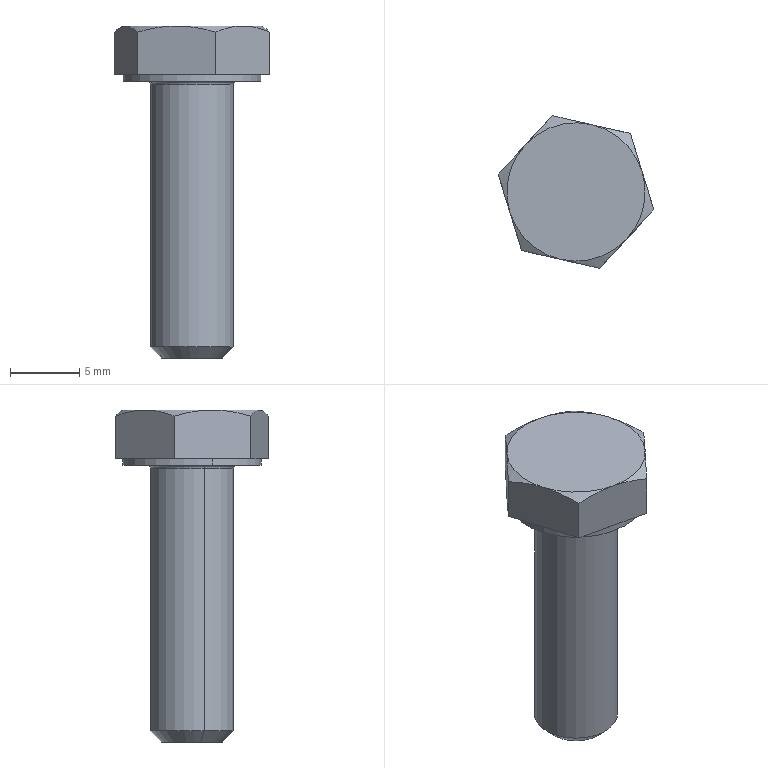Component | SolidWorks | GB_T5781-2000HexHeadBoltFullThreadCGradeM6_20-1 | 1 solid | 29 faces | box 11.25 x 11.04 x 24 mm | volume 902 mm3 | plane 15 | cone 8 | cylinder 4 | torus 2 | commonest cylinder face diameters 6 x2 10 x2 | material 8.8 Grade
STEP:
#1=COLOUR_RGB('',0.7922,0.8196,0.9333);
#2=FILL_AREA_STYLE_COLOUR('',#1);
#3=FILL_AREA_STYLE('',(#2));
#4=SURFACE_STYLE_FILL_AREA(#3);
#5=SURFACE_SIDE_STYLE('',(#4));
#6=SURFACE_STYLE_USAGE(.BOTH.,#5);
#7=PRESENTATION_STYLE_ASSIGNMENT((#6));
#8=CARTESIAN_POINT('',(4.631,0.8511,0.8248));
#9=VERTEX_POINT('',#8);
#10=CARTESIAN_POINT('',(4.857,0.9205,0.8248));
#11=VERTEX_POINT('',#10);
#12=CARTESIAN_POINT('',(4.744,0.8858,0.8248));
#13=DIRECTION('',(0.,0.,-1.));
#14=DIRECTION('',(0.9559,0.2937,0.));
#15=AXIS2_PLACEMENT_3D('',#12,#13,#14);
#16=CIRCLE('',#15,0.1181);
#17=EDGE_CURVE('',#9,#11,#16,.T.);
#18=ORIENTED_EDGE('',*,*,#17,.F.);
#19=CARTESIAN_POINT('',(4.622,0.8482,0.8346));
#20=VERTEX_POINT('',#19);
#21=CARTESIAN_POINT('',(4.622,0.8482,0.8248));
#22=DIRECTION('',(0.2937,-0.9559,0.));
#23=DIRECTION('',(0.9559,0.2937,0.));
#24=AXIS2_PLACEMENT_3D('',#21,#22,#23);
#25=CIRCLE('',#24,0.009843);
#26=EDGE_CURVE('',#9,#20,#25,.T.);
#27=ORIENTED_EDGE('',*,*,#26,.T.);
#28=CARTESIAN_POINT('',(4.866,0.9234,0.8346));
#29=VERTEX_POINT('',#28);
#30=CARTESIAN_POINT('',(4.744,0.8858,0.8346));
#31=DIRECTION('',(0.,0.,1.));
#32=DIRECTION('',(0.9559,0.2937,0.));
#33=AXIS2_PLACEMENT_3D('',#30,#31,#32);
#34=CIRCLE('',#33,0.128);
#35=EDGE_CURVE('',#29,#20,#34,.T.);
#36=ORIENTED_EDGE('',*,*,#35,.F.);
#37=CARTESIAN_POINT('',(4.866,0.9234,0.8248));
#38=DIRECTION('',(-0.2937,0.9559,0.));
#39=DIRECTION('',(-0.9559,-0.2937,0.));
#40=AXIS2_PLACEMENT_3D('',#37,#38,#39);
#41=CIRCLE('',#40,0.009843);
#42=EDGE_CURVE('',#11,#29,#41,.T.);
#43=ORIENTED_EDGE('',*,*,#42,.F.);
#44=EDGE_LOOP('',(#18,#27,#36,#43));
#45=FACE_OUTER_BOUND('',#44,.T.);
#46=CARTESIAN_POINT('',(4.744,0.8858,0.8248));
#47=DIRECTION('',(0.,0.,-1.));
#48=DIRECTION('',(0.9559,0.2937,0.));
#49=AXIS2_PLACEMENT_3D('',#46,#47,#48);
#50=TOROIDAL_SURFACE('',#49,0.128,0.009843);
#51=ADVANCED_FACE('',(#45),#50,.F.);
#52=CARTESIAN_POINT('',(4.827,0.9113,0.04724));
#53=VERTEX_POINT('',#52);
#54=CARTESIAN_POINT('',(4.661,0.8604,0.04724));
#55=VERTEX_POINT('',#54);
#56=CARTESIAN_POINT('',(4.744,0.8858,0.04724));
#57=DIRECTION('',(0.,0.,-1.));
#58=DIRECTION('',(-0.9559,-0.2937,0.));
#59=AXIS2_PLACEMENT_3D('',#56,#57,#58);
#60=CIRCLE('',#59,0.08661);
#61=EDGE_CURVE('',#53,#55,#60,.T.);
#62=ORIENTED_EDGE('',*,*,#61,.F.);
#63=CARTESIAN_POINT('',(4.857,0.9205,0.07874));
#64=VERTEX_POINT('',#63);
#65=CARTESIAN_POINT('',(4.857,0.9205,0.07874));
#66=DIRECTION('',(0.6759,0.2077,0.7071));
#67=VECTOR('',#66,39.37);
#68=LINE('',#65,#67);
#69=EDGE_CURVE('',#53,#64,#68,.T.);
#70=ORIENTED_EDGE('',*,*,#69,.T.);
#71=CARTESIAN_POINT('',(4.631,0.8511,0.07874));
#72=VERTEX_POINT('',#71);
#73=CARTESIAN_POINT('',(4.744,0.8858,0.07874));
#74=DIRECTION('',(0.,0.,1.));
#75=DIRECTION('',(-0.9559,-0.2937,0.));
#76=AXIS2_PLACEMENT_3D('',#73,#74,#75);
#77=CIRCLE('',#76,0.1181);
#78=EDGE_CURVE('',#72,#64,#77,.T.);
#79=ORIENTED_EDGE('',*,*,#78,.F.);
#80=CARTESIAN_POINT('',(4.631,0.8511,0.07874));
#81=DIRECTION('',(-0.6759,-0.2077,0.7071));
#82=VECTOR('',#81,39.37);
#83=LINE('',#80,#82);
#84=EDGE_CURVE('',#55,#72,#83,.T.);
#85=ORIENTED_EDGE('',*,*,#84,.F.);
#86=EDGE_LOOP('',(#62,#70,#79,#85));
#87=FACE_OUTER_BOUND('',#86,.T.);
#88=CARTESIAN_POINT('',(4.744,0.8858,0.07874));
#89=DIRECTION('',(0.,0.,1.));
#90=DIRECTION('',(-0.9559,-0.2937,0.));
#91=AXIS2_PLACEMENT_3D('',#88,#89,#90);
#92=CONICAL_SURFACE('',#91,0.1181,0.7854);
#93=ADVANCED_FACE('',(#87),#92,.T.);
#94=ORIENTED_EDGE('',*,*,#78,.T.);
#95=CARTESIAN_POINT('',(4.857,0.9205,0.9921));
#96=DIRECTION('',(0.,0.,1.));
#97=VECTOR('',#96,39.37);
#98=LINE('',#95,#97);
#99=EDGE_CURVE('',#64,#11,#98,.T.);
#100=ORIENTED_EDGE('',*,*,#99,.T.);
#101=CARTESIAN_POINT('',(4.744,0.8858,0.8248));
#102=DIRECTION('',(0.,0.,-1.));
#103=DIRECTION('',(0.9559,0.2937,0.));
#104=AXIS2_PLACEMENT_3D('',#101,#102,#103);
#105=CIRCLE('',#104,0.1181);
#106=EDGE_CURVE('',#11,#9,#105,.T.);
#107=ORIENTED_EDGE('',*,*,#106,.T.);
#108=CARTESIAN_POINT('',(4.631,0.8511,0.9921));
#109=DIRECTION('',(0.,0.,1.));
#110=VECTOR('',#109,39.37);
#111=LINE('',#108,#110);
#112=EDGE_CURVE('',#72,#9,#111,.T.);
#113=ORIENTED_EDGE('',*,*,#112,.F.);
#114=EDGE_LOOP('',(#94,#100,#107,#113));
#115=FACE_OUTER_BOUND('',#114,.T.);
#116=CARTESIAN_POINT('',(4.744,0.8858,0.9921));
#117=DIRECTION('',(0.,0.,1.));
#118=DIRECTION('',(-0.9559,-0.2937,0.));
#119=AXIS2_PLACEMENT_3D('',#116,#117,#118);
#120=CYLINDRICAL_SURFACE('',#119,0.1181);
#121=ADVANCED_FACE('',(#115),#120,.T.);
#122=CARTESIAN_POINT('',(4.932,0.9436,0.8346));
#123=VERTEX_POINT('',#122);
#124=CARTESIAN_POINT('',(4.556,0.828,0.8346));
#125=VERTEX_POINT('',#124);
#126=CARTESIAN_POINT('',(4.744,0.8858,0.8346));
#127=DIRECTION('',(0.,0.,-1.));
#128=DIRECTION('',(0.9559,0.2937,0.));
#129=AXIS2_PLACEMENT_3D('',#126,#127,#128);
#130=CIRCLE('',#129,0.1969);
#131=EDGE_CURVE('',#123,#125,#130,.T.);
#132=ORIENTED_EDGE('',*,*,#131,.F.);
#133=CARTESIAN_POINT('',(4.932,0.9436,0.8543));
#134=VERTEX_POINT('',#133);
#135=CARTESIAN_POINT('',(4.932,0.9436,0.9921));
#136=DIRECTION('',(0.,0.,1.));
#137=VECTOR('',#136,39.37);
#138=LINE('',#135,#137);
#139=EDGE_CURVE('',#123,#134,#138,.T.);
#140=ORIENTED_EDGE('',*,*,#139,.T.);
#141=CARTESIAN_POINT('',(4.888,0.7518,0.8543));
#142=VERTEX_POINT('',#141);
#143=CARTESIAN_POINT('',(4.744,0.8858,0.8543));
#144=DIRECTION('',(0.,0.,1.));
#145=DIRECTION('',(-0.9559,-0.2937,0.));
#146=AXIS2_PLACEMENT_3D('',#143,#144,#145);
#147=CIRCLE('',#146,0.1969);
#148=EDGE_CURVE('',#142,#134,#147,.T.);
#149=ORIENTED_EDGE('',*,*,#148,.F.);
#150=CARTESIAN_POINT('',(4.7,0.694,0.8543));
#151=VERTEX_POINT('',#150);
#152=CARTESIAN_POINT('',(4.744,0.8858,0.8543));
#153=DIRECTION('',(0.,0.,1.));
#154=DIRECTION('',(-0.9559,-0.2937,0.));
#155=AXIS2_PLACEMENT_3D('',#152,#153,#154);
#156=CIRCLE('',#155,0.1969);
#157=EDGE_CURVE('',#151,#142,#156,.T.);
#158=ORIENTED_EDGE('',*,*,#157,.F.);
#159=CARTESIAN_POINT('',(4.556,0.828,0.8543));
#160=VERTEX_POINT('',#159);
#161=CARTESIAN_POINT('',(4.744,0.8858,0.8543));
#162=DIRECTION('',(0.,0.,1.));
#163=DIRECTION('',(-0.9559,-0.2937,0.));
#164=AXIS2_PLACEMENT_3D('',#161,#162,#163);
#165=CIRCLE('',#164,0.1969);
#166=EDGE_CURVE('',#160,#151,#165,.T.);
#167=ORIENTED_EDGE('',*,*,#166,.F.);
#168=CARTESIAN_POINT('',(4.556,0.828,0.9921));
#169=DIRECTION('',(0.,0.,1.));
#170=VECTOR('',#169,39.37);
#171=LINE('',#168,#170);
#172=EDGE_CURVE('',#125,#160,#171,.T.);
#173=ORIENTED_EDGE('',*,*,#172,.F.);
#174=EDGE_LOOP('',(#132,#140,#149,#158,#167,#173));
#175=FACE_OUTER_BOUND('',#174,.T.);
#176=CARTESIAN_POINT('',(4.744,0.8858,0.9921));
#177=DIRECTION('',(0.,0.,1.));
#178=DIRECTION('',(-0.9559,-0.2937,0.));
#179=AXIS2_PLACEMENT_3D('',#176,#177,#178);
#180=CYLINDRICAL_SURFACE('',#179,0.1969);
#181=ADVANCED_FACE('',(#175),#180,.T.);
#182=CARTESIAN_POINT('',(4.965,0.835,0.8543));
#183=VERTEX_POINT('',#182);
#184=CARTESIAN_POINT('',(4.965,0.835,0.8543));
#185=DIRECTION('',(-0.681,-0.7323,0.));
#186=VECTOR('',#185,39.37);
#187=LINE('',#184,#186);
#188=EDGE_CURVE('',#183,#142,#187,.T.);
#189=ORIENTED_EDGE('',*,*,#188,.F.);
#190=CARTESIAN_POINT('',(4.965,0.835,0.9745));
#191=VERTEX_POINT('',#190);
#192=CARTESIAN_POINT('',(4.965,0.835,0.8346));
#193=DIRECTION('',(0.,0.,1.));
#194=VECTOR('',#193,39.37);
#195=LINE('',#192,#194);
#196=EDGE_CURVE('',#183,#191,#195,.T.);
#197=ORIENTED_EDGE('',*,*,#196,.T.);
#198=CARTESIAN_POINT('',(4.888,0.7518,0.9921));
#199=VERTEX_POINT('',#198);
#200=CARTESIAN_POINT('',(4.888,0.7518,0.9921));
#201=CARTESIAN_POINT('',(4.895,0.7588,0.9921));
#202=CARTESIAN_POINT('',(4.901,0.7659,0.9917));
#203=CARTESIAN_POINT('',(4.914,0.78,0.9901));
#204=CARTESIAN_POINT('',(4.921,0.7869,0.9889));
#205=CARTESIAN_POINT('',(4.94,0.8077,0.9843));
#206=CARTESIAN_POINT('',(4.953,0.8214,0.9799));
#207=CARTESIAN_POINT('',(4.965,0.835,0.9745));
#208=B_SPLINE_CURVE_WITH_KNOTS('',3,(#200,#201,#202,#203,#204,#205,#206,#207),.UNSPECIFIED.,.F.,.F.,(4,2,2,4),(0.002921,0.003649,0.004376,0.005831),.UNSPECIFIED.);
#209=EDGE_CURVE('',#199,#191,#208,.T.);
#210=ORIENTED_EDGE('',*,*,#209,.F.);
#211=CARTESIAN_POINT('',(4.811,0.6686,0.9745));
#212=VERTEX_POINT('',#211);
#213=CARTESIAN_POINT('',(4.811,0.6686,0.9745));
#214=CARTESIAN_POINT('',(4.836,0.6958,0.9853));
#215=CARTESIAN_POINT('',(4.862,0.7234,0.9921));
#216=CARTESIAN_POINT('',(4.888,0.7518,0.9921));
#217=B_SPLINE_CURVE_WITH_KNOTS('',3,(#213,#214,#215,#216),.UNSPECIFIED.,.F.,.F.,(4,4),(0.00000024,0.002921),.UNSPECIFIED.);
#218=EDGE_CURVE('',#212,#199,#217,.T.);
#219=ORIENTED_EDGE('',*,*,#218,.F.);
#220=CARTESIAN_POINT('',(4.811,0.6686,0.8543));
#221=VERTEX_POINT('',#220);
#222=CARTESIAN_POINT('',(4.811,0.6686,0.8346));
#223=DIRECTION('',(0.,0.,1.));
#224=VECTOR('',#223,39.37);
#225=LINE('',#222,#224);
#226=EDGE_CURVE('',#221,#212,#225,.T.);
#227=ORIENTED_EDGE('',*,*,#226,.F.);
#228=CARTESIAN_POINT('',(4.965,0.835,0.8543));
#229=DIRECTION('',(-0.681,-0.7323,0.));
#230=VECTOR('',#229,39.37);
#231=LINE('',#228,#230);
#232=EDGE_CURVE('',#142,#221,#231,.T.);
#233=ORIENTED_EDGE('',*,*,#232,.F.);
#234=EDGE_LOOP('',(#189,#197,#210,#219,#227,#233));
#235=FACE_OUTER_BOUND('',#234,.T.);
#236=CARTESIAN_POINT('',(4.965,0.835,0.8346));
#237=DIRECTION('',(-0.7323,0.681,0.));
#238=DIRECTION('',(0.681,0.7323,0.));
#239=AXIS2_PLACEMENT_3D('',#236,#237,#238);
#240=PLANE('',#239);
#241=ADVANCED_FACE('',(#235),#240,.F.);
#242=CARTESIAN_POINT('',(4.811,0.6686,0.8543));
#243=DIRECTION('',(-0.9747,0.2236,0.));
#244=VECTOR('',#243,39.37);
#245=LINE('',#242,#244);
#246=EDGE_CURVE('',#221,#151,#245,.T.);
#247=ORIENTED_EDGE('',*,*,#246,.F.);
#248=ORIENTED_EDGE('',*,*,#226,.T.);
#249=CARTESIAN_POINT('',(4.7,0.694,0.9921));
#250=VERTEX_POINT('',#249);
#251=CARTESIAN_POINT('',(4.7,0.694,0.9921));
#252=CARTESIAN_POINT('',(4.709,0.6918,0.9921));
#253=CARTESIAN_POINT('',(4.719,0.6896,0.9917));
#254=CARTESIAN_POINT('',(4.737,0.6854,0.9901));
#255=CARTESIAN_POINT('',(4.747,0.6832,0.9889));
#256=CARTESIAN_POINT('',(4.774,0.6769,0.9843));
#257=CARTESIAN_POINT('',(4.793,0.6727,0.9799));
#258=CARTESIAN_POINT('',(4.811,0.6686,0.9745));
#259=B_SPLINE_CURVE_WITH_KNOTS('',3,(#251,#252,#253,#254,#255,#256,#257,#258),.UNSPECIFIED.,.F.,.F.,(4,2,2,4),(0.002921,0.003649,0.004376,0.005831),.UNSPECIFIED.);
#260=EDGE_CURVE('',#250,#212,#259,.T.);
#261=ORIENTED_EDGE('',*,*,#260,.F.);
#262=CARTESIAN_POINT('',(4.589,0.7194,0.9745));
#263=VERTEX_POINT('',#262);
#264=CARTESIAN_POINT('',(4.589,0.7194,0.9745));
#265=CARTESIAN_POINT('',(4.625,0.7111,0.9853));
#266=CARTESIAN_POINT('',(4.662,0.7026,0.9921));
#267=CARTESIAN_POINT('',(4.7,0.694,0.9921));
#268=B_SPLINE_CURVE_WITH_KNOTS('',3,(#264,#265,#266,#267),.UNSPECIFIED.,.F.,.F.,(4,4),(0.00000024,0.002921),.UNSPECIFIED.);
#269=EDGE_CURVE('',#263,#250,#268,.T.);
#270=ORIENTED_EDGE('',*,*,#269,.F.);
#271=CARTESIAN_POINT('',(4.589,0.7194,0.8543));
#272=VERTEX_POINT('',#271);
#273=CARTESIAN_POINT('',(4.589,0.7194,0.8346));
#274=DIRECTION('',(0.,0.,1.));
#275=VECTOR('',#274,39.37);
#276=LINE('',#273,#275);
#277=EDGE_CURVE('',#272,#263,#276,.T.);
#278=ORIENTED_EDGE('',*,*,#277,.F.);
#279=CARTESIAN_POINT('',(4.811,0.6686,0.8543));
#280=DIRECTION('',(-0.9747,0.2236,0.));
#281=VECTOR('',#280,39.37);
#282=LINE('',#279,#281);
#283=EDGE_CURVE('',#151,#272,#282,.T.);
#284=ORIENTED_EDGE('',*,*,#283,.F.);
#285=EDGE_LOOP('',(#247,#248,#261,#270,#278,#284));
#286=FACE_OUTER_BOUND('',#285,.T.);
#287=CARTESIAN_POINT('',(4.811,0.6686,0.8346));
#288=DIRECTION('',(0.2236,0.9747,0.));
#289=DIRECTION('',(0.9747,-0.2236,0.));
#290=AXIS2_PLACEMENT_3D('',#287,#288,#289);
#291=PLANE('',#290);
#292=ADVANCED_FACE('',(#286),#291,.F.);
#293=CARTESIAN_POINT('',(4.589,0.7194,0.8543));
#294=DIRECTION('',(-0.2937,0.9559,0.));
#295=VECTOR('',#294,39.37);
#296=LINE('',#293,#295);
#297=EDGE_CURVE('',#272,#160,#296,.T.);
#298=ORIENTED_EDGE('',*,*,#297,.F.);
#299=ORIENTED_EDGE('',*,*,#277,.T.);
#300=CARTESIAN_POINT('',(4.556,0.828,0.9921));
#301=VERTEX_POINT('',#300);
#302=CARTESIAN_POINT('',(4.556,0.828,0.9921));
#303=CARTESIAN_POINT('',(4.561,0.8096,0.9921));
#304=CARTESIAN_POINT('',(4.567,0.791,0.9904));
#305=CARTESIAN_POINT('',(4.578,0.7547,0.9843));
#306=CARTESIAN_POINT('',(4.584,0.7369,0.9799));
#307=CARTESIAN_POINT('',(4.589,0.7194,0.9745));
#308=B_SPLINE_CURVE_WITH_KNOTS('',3,(#302,#303,#304,#305,#306,#307),.UNSPECIFIED.,.F.,.F.,(4,2,4),(0.008262,0.009724,0.01119),.UNSPECIFIED.);
#309=EDGE_CURVE('',#301,#263,#308,.T.);
#310=ORIENTED_EDGE('',*,*,#309,.F.);
#311=CARTESIAN_POINT('',(4.522,0.9366,0.9745));
#312=VERTEX_POINT('',#311);
#313=CARTESIAN_POINT('',(4.522,0.9366,0.9745));
#314=CARTESIAN_POINT('',(4.528,0.919,0.9799));
#315=CARTESIAN_POINT('',(4.533,0.9009,0.9844));
#316=CARTESIAN_POINT('',(4.544,0.8646,0.9905));
#317=CARTESIAN_POINT('',(4.55,0.8464,0.9921));
#318=CARTESIAN_POINT('',(4.556,0.828,0.9921));
#319=B_SPLINE_CURVE_WITH_KNOTS('',3,(#313,#314,#315,#316,#317,#318),.UNSPECIFIED.,.F.,.F.,(4,2,4),(0.00534,0.006801,0.008262),.UNSPECIFIED.);
#320=EDGE_CURVE('',#312,#301,#319,.T.);
#321=ORIENTED_EDGE('',*,*,#320,.F.);
#322=CARTESIAN_POINT('',(4.522,0.9366,0.8543));
#323=VERTEX_POINT('',#322);
#324=CARTESIAN_POINT('',(4.522,0.9366,0.8346));
#325=DIRECTION('',(0.,0.,1.));
#326=VECTOR('',#325,39.37);
#327=LINE('',#324,#326);
#328=EDGE_CURVE('',#323,#312,#327,.T.);
#329=ORIENTED_EDGE('',*,*,#328,.F.);
#330=CARTESIAN_POINT('',(4.589,0.7194,0.8543));
#331=DIRECTION('',(-0.2937,0.9559,0.));
#332=VECTOR('',#331,39.37);
#333=LINE('',#330,#332);
#334=EDGE_CURVE('',#160,#323,#333,.T.);
#335=ORIENTED_EDGE('',*,*,#334,.F.);
#336=EDGE_LOOP('',(#298,#299,#310,#321,#329,#335));
#337=FACE_OUTER_BOUND('',#336,.T.);
#338=CARTESIAN_POINT('',(4.589,0.7194,0.8346));
#339=DIRECTION('',(0.9559,0.2937,0.));
#340=DIRECTION('',(0.2937,-0.9559,0.));
#341=AXIS2_PLACEMENT_3D('',#338,#339,#340);
#342=PLANE('',#341);
#343=ADVANCED_FACE('',(#337),#342,.F.);
#344=CARTESIAN_POINT('',(4.6,1.02,0.8543));
#345=VERTEX_POINT('',#344);
#346=CARTESIAN_POINT('',(4.677,1.103,0.8543));
#347=DIRECTION('',(0.681,0.7323,0.));
#348=VECTOR('',#347,39.37);
#349=LINE('',#346,#348);
#350=EDGE_CURVE('',#323,#345,#349,.T.);
#351=ORIENTED_EDGE('',*,*,#350,.F.);
#352=ORIENTED_EDGE('',*,*,#328,.T.);
#353=CARTESIAN_POINT('',(4.6,1.02,0.9921));
#354=VERTEX_POINT('',#353);
#355=CARTESIAN_POINT('',(4.6,1.02,0.9921));
#356=CARTESIAN_POINT('',(4.593,1.013,0.9921));
#357=CARTESIAN_POINT('',(4.587,1.006,0.9917));
#358=CARTESIAN_POINT('',(4.573,0.9917,0.9901));
#359=CARTESIAN_POINT('',(4.567,0.9847,0.9889));
#360=CARTESIAN_POINT('',(4.548,0.9639,0.9843));
#361=CARTESIAN_POINT('',(4.535,0.9502,0.9799));
#362=CARTESIAN_POINT('',(4.522,0.9366,0.9745));
#363=B_SPLINE_CURVE_WITH_KNOTS('',3,(#355,#356,#357,#358,#359,#360,#361,#362),.UNSPECIFIED.,.F.,.F.,(4,2,2,4),(0.002921,0.003649,0.004376,0.005831),.UNSPECIFIED.);
#364=EDGE_CURVE('',#354,#312,#363,.T.);
#365=ORIENTED_EDGE('',*,*,#364,.F.);
#366=CARTESIAN_POINT('',(4.677,1.103,0.9745));
#367=VERTEX_POINT('',#366);
#368=CARTESIAN_POINT('',(4.677,1.103,0.9745));
#369=CARTESIAN_POINT('',(4.652,1.076,0.9853));
#370=CARTESIAN_POINT('',(4.626,1.048,0.9921));
#371=CARTESIAN_POINT('',(4.6,1.02,0.9921));
#372=B_SPLINE_CURVE_WITH_KNOTS('',3,(#368,#369,#370,#371),.UNSPECIFIED.,.F.,.F.,(4,4),(0.00000024,0.002921),.UNSPECIFIED.);
#373=EDGE_CURVE('',#367,#354,#372,.T.);
#374=ORIENTED_EDGE('',*,*,#373,.F.);
#375=CARTESIAN_POINT('',(4.677,1.103,0.8543));
#376=VERTEX_POINT('',#375);
#377=CARTESIAN_POINT('',(4.677,1.103,0.8346));
#378=DIRECTION('',(0.,0.,1.));
#379=VECTOR('',#378,39.37);
#380=LINE('',#377,#379);
#381=EDGE_CURVE('',#376,#367,#380,.T.);
#382=ORIENTED_EDGE('',*,*,#381,.F.);
#383=CARTESIAN_POINT('',(4.677,1.103,0.8543));
#384=DIRECTION('',(0.681,0.7323,0.));
#385=VECTOR('',#384,39.37);
#386=LINE('',#383,#385);
#387=EDGE_CURVE('',#345,#376,#386,.T.);
#388=ORIENTED_EDGE('',*,*,#387,.F.);
#389=EDGE_LOOP('',(#351,#352,#365,#374,#382,#388));
#390=FACE_OUTER_BOUND('',#389,.T.);
#391=CARTESIAN_POINT('',(4.677,1.103,0.8346));
#392=DIRECTION('',(0.7323,-0.681,0.));
#393=DIRECTION('',(-0.681,-0.7323,0.));
#394=AXIS2_PLACEMENT_3D('',#391,#392,#393);
#395=PLANE('',#394);
#396=ADVANCED_FACE('',(#390),#395,.F.);
#397=CARTESIAN_POINT('',(4.788,1.078,0.8543));
#398=VERTEX_POINT('',#397);
#399=CARTESIAN_POINT('',(4.899,1.052,0.8543));
#400=DIRECTION('',(0.9747,-0.2236,0.));
#401=VECTOR('',#400,39.37);
#402=LINE('',#399,#401);
#403=EDGE_CURVE('',#376,#398,#402,.T.);
#404=ORIENTED_EDGE('',*,*,#403,.F.);
#405=ORIENTED_EDGE('',*,*,#381,.T.);
#406=CARTESIAN_POINT('',(4.788,1.078,0.9921));
#407=VERTEX_POINT('',#406);
#408=CARTESIAN_POINT('',(4.788,1.078,0.9921));
#409=CARTESIAN_POINT('',(4.778,1.08,0.9921));
#410=CARTESIAN_POINT('',(4.769,1.082,0.9917));
#411=CARTESIAN_POINT('',(4.75,1.086,0.9901));
#412=CARTESIAN_POINT('',(4.741,1.088,0.9889));
#413=CARTESIAN_POINT('',(4.713,1.095,0.9843));
#414=CARTESIAN_POINT('',(4.695,1.099,0.9799));
#415=CARTESIAN_POINT('',(4.677,1.103,0.9745));
#416=B_SPLINE_CURVE_WITH_KNOTS('',3,(#408,#409,#410,#411,#412,#413,#414,#415),.UNSPECIFIED.,.F.,.F.,(4,2,2,4),(0.002921,0.003649,0.004376,0.005831),.UNSPECIFIED.);
#417=EDGE_CURVE('',#407,#367,#416,.T.);
#418=ORIENTED_EDGE('',*,*,#417,.F.);
#419=CARTESIAN_POINT('',(4.899,1.052,0.9745));
#420=VERTEX_POINT('',#419);
#421=CARTESIAN_POINT('',(4.899,1.052,0.9745));
#422=CARTESIAN_POINT('',(4.862,1.061,0.9853));
#423=CARTESIAN_POINT('',(4.826,1.069,0.9921));
#424=CARTESIAN_POINT('',(4.788,1.078,0.9921));
#425=B_SPLINE_CURVE_WITH_KNOTS('',3,(#421,#422,#423,#424),.UNSPECIFIED.,.F.,.F.,(4,4),(0.00000024,0.002921),.UNSPECIFIED.);
#426=EDGE_CURVE('',#420,#407,#425,.T.);
#427=ORIENTED_EDGE('',*,*,#426,.F.);
#428=CARTESIAN_POINT('',(4.899,1.052,0.8543));
#429=VERTEX_POINT('',#428);
#430=CARTESIAN_POINT('',(4.899,1.052,0.8346));
#431=DIRECTION('',(0.,0.,1.));
#432=VECTOR('',#431,39.37);
#433=LINE('',#430,#432);
#434=EDGE_CURVE('',#429,#420,#433,.T.);
#435=ORIENTED_EDGE('',*,*,#434,.F.);
#436=CARTESIAN_POINT('',(4.899,1.052,0.8543));
#437=DIRECTION('',(0.9747,-0.2236,0.));
#438=VECTOR('',#437,39.37);
#439=LINE('',#436,#438);
#440=EDGE_CURVE('',#398,#429,#439,.T.);
#441=ORIENTED_EDGE('',*,*,#440,.F.);
#442=EDGE_LOOP('',(#404,#405,#418,#427,#435,#441));
#443=FACE_OUTER_BOUND('',#442,.T.);
#444=CARTESIAN_POINT('',(4.899,1.052,0.8346));
#445=DIRECTION('',(-0.2236,-0.9747,0.));
#446=DIRECTION('',(-0.9747,0.2236,0.));
#447=AXIS2_PLACEMENT_3D('',#444,#445,#446);
#448=PLANE('',#447);
#449=ADVANCED_FACE('',(#443),#448,.F.);
#450=CARTESIAN_POINT('',(4.965,0.835,0.8543));
#451=DIRECTION('',(0.2937,-0.9559,0.));
#452=VECTOR('',#451,39.37);
#453=LINE('',#450,#452);
#454=EDGE_CURVE('',#429,#134,#453,.T.);
#455=ORIENTED_EDGE('',*,*,#454,.F.);
#456=ORIENTED_EDGE('',*,*,#434,.T.);
#457=CARTESIAN_POINT('',(4.932,0.9436,0.9921));
#458=VERTEX_POINT('',#457);
#459=CARTESIAN_POINT('',(4.932,0.9436,0.9921));
#460=CARTESIAN_POINT('',(4.926,0.962,0.9921));
#461=CARTESIAN_POINT('',(4.921,0.9803,0.9905));
#462=CARTESIAN_POINT('',(4.91,1.017,0.9844));
#463=CARTESIAN_POINT('',(4.904,1.035,0.9799));
#464=CARTESIAN_POINT('',(4.899,1.052,0.9745));
#465=B_SPLINE_CURVE_WITH_KNOTS('',3,(#459,#460,#461,#462,#463,#464),.UNSPECIFIED.,.F.,.F.,(4,2,4),(0.01799,0.01945,0.02091),.UNSPECIFIED.);
#466=EDGE_CURVE('',#458,#420,#465,.T.);
#467=ORIENTED_EDGE('',*,*,#466,.F.);
#468=CARTESIAN_POINT('',(4.965,0.835,0.9745));
#469=CARTESIAN_POINT('',(4.96,0.8526,0.9799));
#470=CARTESIAN_POINT('',(4.955,0.8704,0.9843));
#471=CARTESIAN_POINT('',(4.943,0.9066,0.9904));
#472=CARTESIAN_POINT('',(4.938,0.9253,0.9921));
#473=CARTESIAN_POINT('',(4.932,0.9436,0.9921));
#474=B_SPLINE_CURVE_WITH_KNOTS('',3,(#468,#469,#470,#471,#472,#473),.UNSPECIFIED.,.F.,.F.,(4,2,4),(0.01507,0.01653,0.01799),.UNSPECIFIED.);
#475=EDGE_CURVE('',#191,#458,#474,.T.);
#476=ORIENTED_EDGE('',*,*,#475,.F.);
#477=ORIENTED_EDGE('',*,*,#196,.F.);
#478=CARTESIAN_POINT('',(4.965,0.835,0.8543));
#479=DIRECTION('',(0.2937,-0.9559,0.));
#480=VECTOR('',#479,39.37);
#481=LINE('',#478,#480);
#482=EDGE_CURVE('',#134,#183,#481,.T.);
#483=ORIENTED_EDGE('',*,*,#482,.F.);
#484=EDGE_LOOP('',(#455,#456,#467,#476,#477,#483));
#485=FACE_OUTER_BOUND('',#484,.T.);
#486=CARTESIAN_POINT('',(4.965,0.835,0.8346));
#487=DIRECTION('',(-0.9559,-0.2937,0.));
#488=DIRECTION('',(-0.2937,0.9559,0.));
#489=AXIS2_PLACEMENT_3D('',#486,#487,#488);
#490=PLANE('',#489);
#491=ADVANCED_FACE('',(#485),#490,.F.);
#492=ORIENTED_EDGE('',*,*,#426,.T.);
#493=CARTESIAN_POINT('',(4.744,0.8858,0.9921));
#494=DIRECTION('',(0.,0.,-1.));
#495=DIRECTION('',(0.9559,0.2937,0.));
#496=AXIS2_PLACEMENT_3D('',#493,#494,#495);
#497=CIRCLE('',#496,0.1969);
#498=EDGE_CURVE('',#407,#458,#497,.T.);
#499=ORIENTED_EDGE('',*,*,#498,.T.);
#500=ORIENTED_EDGE('',*,*,#466,.T.);
#501=EDGE_LOOP('',(#492,#499,#500));
#502=FACE_OUTER_BOUND('',#501,.T.);
#503=CARTESIAN_POINT('',(4.744,0.8858,0.9921));
#504=DIRECTION('',(0.,0.,-1.));
#505=DIRECTION('',(0.9559,0.2937,0.));
#506=AXIS2_PLACEMENT_3D('',#503,#504,#505);
#507=CONICAL_SURFACE('',#506,0.1969,1.047);
#508=ADVANCED_FACE('',(#502),#507,.T.);
#509=ORIENTED_EDGE('',*,*,#373,.T.);
#510=CARTESIAN_POINT('',(4.744,0.8858,0.9921));
#511=DIRECTION('',(0.,0.,-1.));
#512=DIRECTION('',(0.9559,0.2937,0.));
#513=AXIS2_PLACEMENT_3D('',#510,#511,#512);
#514=CIRCLE('',#513,0.1969);
#515=EDGE_CURVE('',#354,#407,#514,.T.);
#516=ORIENTED_EDGE('',*,*,#515,.T.);
#517=ORIENTED_EDGE('',*,*,#417,.T.);
#518=EDGE_LOOP('',(#509,#516,#517));
#519=FACE_OUTER_BOUND('',#518,.T.);
#520=CARTESIAN_POINT('',(4.744,0.8858,0.9921));
#521=DIRECTION('',(0.,0.,-1.));
#522=DIRECTION('',(0.9559,0.2937,0.));
#523=AXIS2_PLACEMENT_3D('',#520,#521,#522);
#524=CONICAL_SURFACE('',#523,0.1969,1.047);
#525=ADVANCED_FACE('',(#519),#524,.T.);
#526=ORIENTED_EDGE('',*,*,#320,.T.);
#527=CARTESIAN_POINT('',(4.744,0.8858,0.9921));
#528=DIRECTION('',(0.,0.,-1.));
#529=DIRECTION('',(0.9559,0.2937,0.));
#530=AXIS2_PLACEMENT_3D('',#527,#528,#529);
#531=CIRCLE('',#530,0.1969);
#532=EDGE_CURVE('',#301,#354,#531,.T.);
#533=ORIENTED_EDGE('',*,*,#532,.T.);
#534=ORIENTED_EDGE('',*,*,#364,.T.);
#535=EDGE_LOOP('',(#526,#533,#534));
#536=FACE_OUTER_BOUND('',#535,.T.);
#537=CARTESIAN_POINT('',(4.744,0.8858,0.9921));
#538=DIRECTION('',(0.,0.,-1.));
#539=DIRECTION('',(0.9559,0.2937,0.));
#540=AXIS2_PLACEMENT_3D('',#537,#538,#539);
#541=CONICAL_SURFACE('',#540,0.1969,1.047);
#542=ADVANCED_FACE('',(#536),#541,.T.);
#543=ORIENTED_EDGE('',*,*,#309,.T.);
#544=ORIENTED_EDGE('',*,*,#269,.T.);
#545=CARTESIAN_POINT('',(4.744,0.8858,0.9921));
#546=DIRECTION('',(0.,0.,1.));
#547=DIRECTION('',(-0.9559,-0.2937,0.));
#548=AXIS2_PLACEMENT_3D('',#545,#546,#547);
#549=CIRCLE('',#548,0.1969);
#550=EDGE_CURVE('',#301,#250,#549,.T.);
#551=ORIENTED_EDGE('',*,*,#550,.F.);
#552=EDGE_LOOP('',(#543,#544,#551));
#553=FACE_OUTER_BOUND('',#552,.T.);
#554=CARTESIAN_POINT('',(4.744,0.8858,0.9921));
#555=DIRECTION('',(0.,0.,-1.));
#556=DIRECTION('',(0.9559,0.2937,0.));
#557=AXIS2_PLACEMENT_3D('',#554,#555,#556);
#558=CONICAL_SURFACE('',#557,0.1969,1.047);
#559=ADVANCED_FACE('',(#553),#558,.T.);
#560=ORIENTED_EDGE('',*,*,#260,.T.);
#561=ORIENTED_EDGE('',*,*,#218,.T.);
#562=CARTESIAN_POINT('',(4.744,0.8858,0.9921));
#563=DIRECTION('',(0.,0.,-1.));
#564=DIRECTION('',(0.9559,0.2937,0.));
#565=AXIS2_PLACEMENT_3D('',#562,#563,#564);
#566=CIRCLE('',#565,0.1969);
#567=EDGE_CURVE('',#199,#250,#566,.T.);
#568=ORIENTED_EDGE('',*,*,#567,.T.);
#569=EDGE_LOOP('',(#560,#561,#568));
#570=FACE_OUTER_BOUND('',#569,.T.);
#571=CARTESIAN_POINT('',(4.744,0.8858,0.9921));
#572=DIRECTION('',(0.,0.,-1.));
#573=DIRECTION('',(0.9559,0.2937,0.));
#574=AXIS2_PLACEMENT_3D('',#571,#572,#573);
#575=CONICAL_SURFACE('',#574,0.1969,1.047);
#576=ADVANCED_FACE('',(#570),#575,.T.);
#577=ORIENTED_EDGE('',*,*,#209,.T.);
#578=ORIENTED_EDGE('',*,*,#475,.T.);
#579=CARTESIAN_POINT('',(4.744,0.8858,0.9921));
#580=DIRECTION('',(0.,0.,-1.));
#581=DIRECTION('',(0.9559,0.2937,0.));
#582=AXIS2_PLACEMENT_3D('',#579,#580,#581);
#583=CIRCLE('',#582,0.1969);
#584=EDGE_CURVE('',#458,#199,#583,.T.);
#585=ORIENTED_EDGE('',*,*,#584,.T.);
#586=EDGE_LOOP('',(#577,#578,#585));
#587=FACE_OUTER_BOUND('',#586,.T.);
#588=CARTESIAN_POINT('',(4.744,0.8858,0.9921));
#589=DIRECTION('',(0.,0.,-1.));
#590=DIRECTION('',(0.9559,0.2937,0.));
#591=AXIS2_PLACEMENT_3D('',#588,#589,#590);
#592=CONICAL_SURFACE('',#591,0.1969,1.047);
#593=ADVANCED_FACE('',(#587),#592,.T.);
#594=ORIENTED_EDGE('',*,*,#584,.F.);
#595=ORIENTED_EDGE('',*,*,#498,.F.);
#596=ORIENTED_EDGE('',*,*,#515,.F.);
#597=ORIENTED_EDGE('',*,*,#532,.F.);
#598=ORIENTED_EDGE('',*,*,#550,.T.);
#599=ORIENTED_EDGE('',*,*,#567,.F.);
#600=EDGE_LOOP('',(#594,#595,#596,#597,#598,#599));
#601=FACE_OUTER_BOUND('',#600,.T.);
#602=CARTESIAN_POINT('',(5.12,1.001,0.9921));
#603=DIRECTION('',(0.,0.,-1.));
#604=DIRECTION('',(0.9559,0.2937,0.));
#605=AXIS2_PLACEMENT_3D('',#602,#603,#604);
#606=PLANE('',#605);
#607=ADVANCED_FACE('',(#601),#606,.F.);
#608=ORIENTED_EDGE('',*,*,#188,.T.);
#609=ORIENTED_EDGE('',*,*,#148,.T.);
#610=ORIENTED_EDGE('',*,*,#482,.T.);
#611=EDGE_LOOP('',(#608,#609,#610));
#612=FACE_OUTER_BOUND('',#611,.T.);
#613=CARTESIAN_POINT('',(4.802,0.6977,0.8543));
#614=DIRECTION('',(0.,0.,-1.));
#615=DIRECTION('',(0.9559,0.2937,0.));
#616=AXIS2_PLACEMENT_3D('',#613,#614,#615);
#617=PLANE('',#616);
#618=ADVANCED_FACE('',(#612),#617,.T.);
#619=ORIENTED_EDGE('',*,*,#232,.T.);
#620=ORIENTED_EDGE('',*,*,#246,.T.);
#621=ORIENTED_EDGE('',*,*,#157,.T.);
#622=EDGE_LOOP('',(#619,#620,#621));
#623=FACE_OUTER_BOUND('',#622,.T.);
#624=CARTESIAN_POINT('',(4.802,0.6977,0.8543));
#625=DIRECTION('',(0.,0.,-1.));
#626=DIRECTION('',(0.9559,0.2937,0.));
#627=AXIS2_PLACEMENT_3D('',#624,#625,#626);
#628=PLANE('',#627);
#629=ADVANCED_FACE('',(#623),#628,.T.);
#630=ORIENTED_EDGE('',*,*,#283,.T.);
#631=ORIENTED_EDGE('',*,*,#297,.T.);
#632=ORIENTED_EDGE('',*,*,#166,.T.);
#633=EDGE_LOOP('',(#630,#631,#632));
#634=FACE_OUTER_BOUND('',#633,.T.);
#635=CARTESIAN_POINT('',(4.802,0.6977,0.8543));
#636=DIRECTION('',(0.,0.,-1.));
#637=DIRECTION('',(0.9559,0.2937,0.));
#638=AXIS2_PLACEMENT_3D('',#635,#636,#637);
#639=PLANE('',#638);
#640=ADVANCED_FACE('',(#634),#639,.T.);
#641=ORIENTED_EDGE('',*,*,#334,.T.);
#642=ORIENTED_EDGE('',*,*,#350,.T.);
#643=CARTESIAN_POINT('',(4.744,0.8858,0.8543));
#644=DIRECTION('',(0.,0.,1.));
#645=DIRECTION('',(-0.9559,-0.2937,0.));
#646=AXIS2_PLACEMENT_3D('',#643,#644,#645);
#647=CIRCLE('',#646,0.1969);
#648=EDGE_CURVE('',#345,#160,#647,.T.);
#649=ORIENTED_EDGE('',*,*,#648,.T.);
#650=EDGE_LOOP('',(#641,#642,#649));
#651=FACE_OUTER_BOUND('',#650,.T.);
#652=CARTESIAN_POINT('',(4.802,0.6977,0.8543));
#653=DIRECTION('',(0.,0.,-1.));
#654=DIRECTION('',(0.9559,0.2937,0.));
#655=AXIS2_PLACEMENT_3D('',#652,#653,#654);
#656=PLANE('',#655);
#657=ADVANCED_FACE('',(#651),#656,.T.);
#658=ORIENTED_EDGE('',*,*,#387,.T.);
#659=ORIENTED_EDGE('',*,*,#403,.T.);
#660=CARTESIAN_POINT('',(4.744,0.8858,0.8543));
#661=DIRECTION('',(0.,0.,1.));
#662=DIRECTION('',(-0.9559,-0.2937,0.));
#663=AXIS2_PLACEMENT_3D('',#660,#661,#662);
#664=CIRCLE('',#663,0.1969);
#665=EDGE_CURVE('',#398,#345,#664,.T.);
#666=ORIENTED_EDGE('',*,*,#665,.T.);
#667=EDGE_LOOP('',(#658,#659,#666));
#668=FACE_OUTER_BOUND('',#667,.T.);
#669=CARTESIAN_POINT('',(4.802,0.6977,0.8543));
#670=DIRECTION('',(0.,0.,-1.));
#671=DIRECTION('',(0.9559,0.2937,0.));
#672=AXIS2_PLACEMENT_3D('',#669,#670,#671);
#673=PLANE('',#672);
#674=ADVANCED_FACE('',(#668),#673,.T.);
#675=ORIENTED_EDGE('',*,*,#440,.T.);
#676=ORIENTED_EDGE('',*,*,#454,.T.);
#677=CARTESIAN_POINT('',(4.744,0.8858,0.8543));
#678=DIRECTION('',(0.,0.,1.));
#679=DIRECTION('',(-0.9559,-0.2937,0.));
#680=AXIS2_PLACEMENT_3D('',#677,#678,#679);
#681=CIRCLE('',#680,0.1969);
#682=EDGE_CURVE('',#134,#398,#681,.T.);
#683=ORIENTED_EDGE('',*,*,#682,.T.);
#684=EDGE_LOOP('',(#675,#676,#683));
#685=FACE_OUTER_BOUND('',#684,.T.);
#686=CARTESIAN_POINT('',(4.802,0.6977,0.8543));
#687=DIRECTION('',(0.,0.,-1.));
#688=DIRECTION('',(0.9559,0.2937,0.));
#689=AXIS2_PLACEMENT_3D('',#686,#687,#688);
#690=PLANE('',#689);
#691=ADVANCED_FACE('',(#685),#690,.T.);
#692=ORIENTED_EDGE('',*,*,#139,.F.);
#693=CARTESIAN_POINT('',(4.744,0.8858,0.8346));
#694=DIRECTION('',(0.,0.,-1.));
#695=DIRECTION('',(0.9559,0.2937,0.));
#696=AXIS2_PLACEMENT_3D('',#693,#694,#695);
#697=CIRCLE('',#696,0.1969);
#698=EDGE_CURVE('',#125,#123,#697,.T.);
#699=ORIENTED_EDGE('',*,*,#698,.F.);
#700=ORIENTED_EDGE('',*,*,#172,.T.);
#701=ORIENTED_EDGE('',*,*,#648,.F.);
#702=ORIENTED_EDGE('',*,*,#665,.F.);
#703=ORIENTED_EDGE('',*,*,#682,.F.);
#704=EDGE_LOOP('',(#692,#699,#700,#701,#702,#703));
#705=FACE_OUTER_BOUND('',#704,.T.);
#706=CARTESIAN_POINT('',(4.744,0.8858,0.9921));
#707=DIRECTION('',(0.,0.,1.));
#708=DIRECTION('',(-0.9559,-0.2937,0.));
#709=AXIS2_PLACEMENT_3D('',#706,#707,#708);
#710=CYLINDRICAL_SURFACE('',#709,0.1969);
#711=ADVANCED_FACE('',(#705),#710,.T.);
#712=CARTESIAN_POINT('',(4.744,0.8858,0.04724));
#713=DIRECTION('',(0.,0.,-1.));
#714=DIRECTION('',(-0.9559,-0.2937,0.));
#715=AXIS2_PLACEMENT_3D('',#712,#713,#714);
#716=CIRCLE('',#715,0.08661);
#717=EDGE_CURVE('',#55,#53,#716,.T.);
#718=ORIENTED_EDGE('',*,*,#717,.T.);
#719=ORIENTED_EDGE('',*,*,#61,.T.);
#720=EDGE_LOOP('',(#718,#719));
#721=FACE_OUTER_BOUND('',#720,.T.);
#722=CARTESIAN_POINT('',(4.744,0.8858,0.04724));
#723=DIRECTION('',(0.,0.,1.));
#724=DIRECTION('',(-0.9559,-0.2937,0.));
#725=AXIS2_PLACEMENT_3D('',#722,#723,#724);
#726=PLANE('',#725);
#727=ADVANCED_FACE('',(#721),#726,.F.);
#728=ORIENTED_EDGE('',*,*,#99,.F.);
#729=CARTESIAN_POINT('',(4.744,0.8858,0.07874));
#730=DIRECTION('',(0.,0.,1.));
#731=DIRECTION('',(-0.9559,-0.2937,0.));
#732=AXIS2_PLACEMENT_3D('',#729,#730,#731);
#733=CIRCLE('',#732,0.1181);
#734=EDGE_CURVE('',#64,#72,#733,.T.);
#735=ORIENTED_EDGE('',*,*,#734,.T.);
#736=ORIENTED_EDGE('',*,*,#112,.T.);
#737=ORIENTED_EDGE('',*,*,#17,.T.);
#738=EDGE_LOOP('',(#728,#735,#736,#737));
#739=FACE_OUTER_BOUND('',#738,.T.);
#740=CARTESIAN_POINT('',(4.744,0.8858,0.9921));
#741=DIRECTION('',(0.,0.,1.));
#742=DIRECTION('',(-0.9559,-0.2937,0.));
#743=AXIS2_PLACEMENT_3D('',#740,#741,#742);
#744=CYLINDRICAL_SURFACE('',#743,0.1181);
#745=ADVANCED_FACE('',(#739),#744,.T.);
#746=ORIENTED_EDGE('',*,*,#35,.T.);
#747=CARTESIAN_POINT('',(4.744,0.8858,0.8346));
#748=DIRECTION('',(0.,0.,1.));
#749=DIRECTION('',(0.9559,0.2937,0.));
#750=AXIS2_PLACEMENT_3D('',#747,#748,#749);
#751=CIRCLE('',#750,0.128);
#752=EDGE_CURVE('',#20,#29,#751,.T.);
#753=ORIENTED_EDGE('',*,*,#752,.T.);
#754=EDGE_LOOP('',(#746,#753));
#755=FACE_BOUND('',#754,.T.);
#756=ORIENTED_EDGE('',*,*,#698,.T.);
#757=ORIENTED_EDGE('',*,*,#131,.T.);
#758=EDGE_LOOP('',(#756,#757));
#759=FACE_OUTER_BOUND('',#758,.T.);
#760=CARTESIAN_POINT('',(5.12,1.001,0.8346));
#761=DIRECTION('',(0.,0.,-1.));
#762=DIRECTION('',(0.9559,0.2937,0.));
#763=AXIS2_PLACEMENT_3D('',#760,#761,#762);
#764=PLANE('',#763);
#765=ADVANCED_FACE('',(#755,#759),#764,.T.);
#766=ORIENTED_EDGE('',*,*,#69,.F.);
#767=ORIENTED_EDGE('',*,*,#717,.F.);
#768=ORIENTED_EDGE('',*,*,#84,.T.);
#769=ORIENTED_EDGE('',*,*,#734,.F.);
#770=EDGE_LOOP('',(#766,#767,#768,#769));
#771=FACE_OUTER_BOUND('',#770,.T.);
#772=CARTESIAN_POINT('',(4.744,0.8858,0.07874));
#773=DIRECTION('',(0.,0.,1.));
#774=DIRECTION('',(-0.9559,-0.2937,0.));
#775=AXIS2_PLACEMENT_3D('',#772,#773,#774);
#776=CONICAL_SURFACE('',#775,0.1181,0.7854);
#777=ADVANCED_FACE('',(#771),#776,.T.);
#778=ORIENTED_EDGE('',*,*,#26,.F.);
#779=ORIENTED_EDGE('',*,*,#106,.F.);
#780=ORIENTED_EDGE('',*,*,#42,.T.);
#781=ORIENTED_EDGE('',*,*,#752,.F.);
#782=EDGE_LOOP('',(#778,#779,#780,#781));
#783=FACE_OUTER_BOUND('',#782,.T.);
#784=CARTESIAN_POINT('',(4.744,0.8858,0.8248));
#785=DIRECTION('',(0.,0.,-1.));
#786=DIRECTION('',(0.9559,0.2937,0.));
#787=AXIS2_PLACEMENT_3D('',#784,#785,#786);
#788=TOROIDAL_SURFACE('',#787,0.128,0.009843);
#789=ADVANCED_FACE('',(#783),#788,.F.);
#790=CLOSED_SHELL('',(#51,#93,#121,#181,#241,#292,#343,#396,#449,#491,#508,#525,#542,#559,#576,#593,#607,#618,#629,#640,#657,#674,#691,#711,#727,#745,#765,#777,#789));
#791=MANIFOLD_SOLID_BREP('',#790);
#792=STYLED_ITEM('',(#7),#791);
#793=PRESENTATION_LAYER_ASSIGNMENT('','',(#792));
#794=(LENGTH_UNIT()NAMED_UNIT(*)SI_UNIT($,.METRE.));
#795=LENGTH_MEASURE_WITH_UNIT(LENGTH_MEASURE(0.0254),#794);
#796=DIMENSIONAL_EXPONENTS(1.,0.,0.,0.,0.,0.,0.);
#797=(CONVERSION_BASED_UNIT('',#795)LENGTH_UNIT()NAMED_UNIT(#796));
#798=UNCERTAINTY_MEASURE_WITH_UNIT(LENGTH_MEASURE(0.00001),#797,'','');
#799=(NAMED_UNIT(*)PLANE_ANGLE_UNIT()SI_UNIT($,.RADIAN.));
#800=(NAMED_UNIT(*)SI_UNIT($,.STERADIAN.)SOLID_ANGLE_UNIT());
#801=(GEOMETRIC_REPRESENTATION_CONTEXT(3)GLOBAL_UNCERTAINTY_ASSIGNED_CONTEXT((#798))GLOBAL_UNIT_ASSIGNED_CONTEXT((#797,#799,#800))REPRESENTATION_CONTEXT('',''));
#802=MECHANICAL_DESIGN_GEOMETRIC_PRESENTATION_REPRESENTATION('',(#792),#801);
#803=CARTESIAN_POINT('',(0.,0.,0.));
#804=DIRECTION('',(0.,0.,1.));
#805=DIRECTION('',(1.,0.,0.));
#806=AXIS2_PLACEMENT_3D('',#803,#804,#805);
#807=(LENGTH_UNIT()NAMED_UNIT(*)SI_UNIT($,.METRE.));
#808=LENGTH_MEASURE_WITH_UNIT(LENGTH_MEASURE(0.0254),#807);
#809=DIMENSIONAL_EXPONENTS(1.,0.,0.,0.,0.,0.,0.);
#810=(CONVERSION_BASED_UNIT('',#808)LENGTH_UNIT()NAMED_UNIT(#809));
#811=UNCERTAINTY_MEASURE_WITH_UNIT(LENGTH_MEASURE(0.00001),#810,'','');
#812=(NAMED_UNIT(*)PLANE_ANGLE_UNIT()SI_UNIT($,.RADIAN.));
#813=(NAMED_UNIT(*)SI_UNIT($,.STERADIAN.)SOLID_ANGLE_UNIT());
#814=(GEOMETRIC_REPRESENTATION_CONTEXT(3)GLOBAL_UNCERTAINTY_ASSIGNED_CONTEXT((#811))GLOBAL_UNIT_ASSIGNED_CONTEXT((#810,#812,#813))REPRESENTATION_CONTEXT('',''));
#815=ADVANCED_BREP_SHAPE_REPRESENTATION('',(#791,#806),#814);